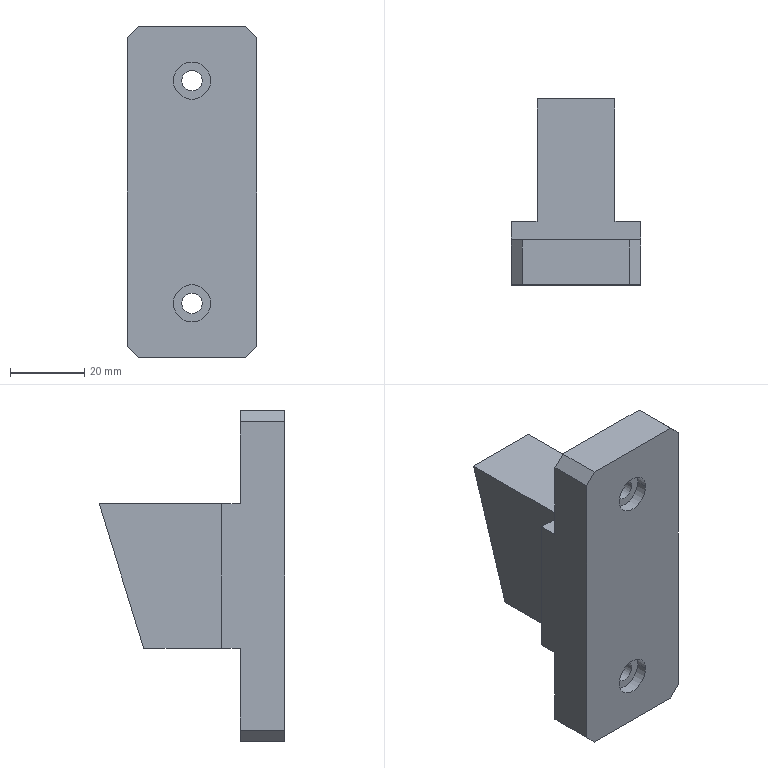Component | SolidWorks | QX1-15-PusherSlider-1 | 1 solid | 32 faces | box 35 x 50 x 89 mm | volume 64993 mm3 | plane 20 | cylinder 8 | cone 4 | commonest cylinder face diameters 5.5 x4 10 x4 | material PA Type 6
build123d program:
from build123d import *

# Parameters (mm, degrees)
BOSS_EXTRUDE1_DEPTH                                  = 17.5
SKETCH2_W                                            = 89
SKETCH2_H                                            = 12
BOSS_EXTRUDE2_DEPTH                                  = 35
SKETCH3_R                                            = 5
CUT_EXTRUDE1_DEPTH                                   = 3
CONICAL_COUNTERSUNK_HOLE1_FOR_M5_HEXAGON_D           = 5.5
CONICAL_COUNTERSUNK_HOLE1_FOR_M5_HEXAGON_CSINK_D     = 11.47
CONICAL_COUNTERSUNK_HOLE1_FOR_M5_HEXAGON_CSINK_ANGLE = 90
SKETCH7_W                                            = 39
SKETCH7_H                                            = 33
CUT_EXTRUDE2_DEPTH                                   = 7
CHAMFER1_SIZE                                        = 3


with BuildPart() as part:
    # Sketch1 → Boss-Extrude1 (new, symmetric)
    with BuildSketch(Plane.XY):
        Polygon((0, 0), (0, 38), (39, 50), (39, 0), align=None)
    extrude(amount=BOSS_EXTRUDE1_DEPTH, both=True)

    # Sketch2 → Boss-Extrude2 (add)
    with BuildSketch(Plane.XY.offset(17.5)):
        with Locations((19.5, 6)):
            Rectangle(SKETCH2_W, SKETCH2_H)
    extrude(amount=-BOSS_EXTRUDE2_DEPTH)

    # Sketch3 → Cut-Extrude1 (cut)
    with BuildSketch(Plane.XZ):
        with Locations(Location((-10.5, 0, 0), (0, 0, 270))):
            Circle(SKETCH3_R)
        with Locations(Location((49.5, 0, 0), (0, 0, 270))):
            Circle(SKETCH3_R)
    extrude(amount=-CUT_EXTRUDE1_DEPTH, mode=Mode.SUBTRACT)

    # Conical Countersunk Hole1 for M5 Hexagon (through all)
    with Locations(Plane(origin=(0, 12, 0), x_dir=(1, 0, 0), z_dir=(0, 1, 0))):
        with Locations((-10.5, 0), (49.5, 0)):
            CounterSinkHole(CONICAL_COUNTERSUNK_HOLE1_FOR_M5_HEXAGON_D / 2, CONICAL_COUNTERSUNK_HOLE1_FOR_M5_HEXAGON_CSINK_D / 2, counter_sink_angle=CONICAL_COUNTERSUNK_HOLE1_FOR_M5_HEXAGON_CSINK_ANGLE)

    # Sketch7 → Cut-Extrude2 (cut)
    with BuildSketch(Plane.XY.offset(17.5)):
        with Locations((19.5, 33.5)):
            Rectangle(SKETCH7_W, SKETCH7_H)
    cut_extrude2 = extrude(amount=-CUT_EXTRUDE2_DEPTH, mode=Mode.SUBTRACT)

    # Mirror1: Cut-Extrude2 across plane
    add(cut_extrude2.mirror(Plane.XY), mode=Mode.SUBTRACT)

    # Chamfer1
    chamfer1_edges = [part.edges().sort_by_distance(p)[0] for p in [
        (64, 6, 17.5),
        (-25, 6, 17.5),
        (-25, 6, -17.5),
        (64, 6, -17.5),
    ]]
    chamfer(chamfer1_edges, length=CHAMFER1_SIZE)


solid = part.part

# Placed as in the assembly
solid = solid.moved(Location((0, 40, -19.5), (0, -90, 0)))
STEP:
#1=COLOUR_RGB('',0.7922,0.8196,0.9333);
#2=FILL_AREA_STYLE_COLOUR('',#1);
#3=FILL_AREA_STYLE('',(#2));
#4=SURFACE_STYLE_FILL_AREA(#3);
#5=SURFACE_SIDE_STYLE('',(#4));
#6=SURFACE_STYLE_USAGE(.BOTH.,#5);
#7=PRESENTATION_STYLE_ASSIGNMENT((#6));
#8=CARTESIAN_POINT('',(0.1083,1.93,-1.181));
#9=VERTEX_POINT('',#8);
#10=CARTESIAN_POINT('',(-0.1083,1.93,-1.181));
#11=VERTEX_POINT('',#10);
#12=CARTESIAN_POINT('',(0.,1.93,-1.181));
#13=DIRECTION('',(-0.,1.,-0.));
#14=DIRECTION('',(-1.,-0.,0.));
#15=AXIS2_PLACEMENT_3D('',#12,#13,#14);
#16=CIRCLE('',#15,0.1083);
#17=EDGE_CURVE('',#9,#11,#16,.T.);
#18=ORIENTED_EDGE('',*,*,#17,.F.);
#19=CARTESIAN_POINT('',(0.2258,2.047,-1.181));
#20=VERTEX_POINT('',#19);
#21=CARTESIAN_POINT('',(0.2258,2.047,-1.181));
#22=DIRECTION('',(0.7071,0.7071,0.));
#23=VECTOR('',#22,39.37);
#24=LINE('',#21,#23);
#25=EDGE_CURVE('',#9,#20,#24,.T.);
#26=ORIENTED_EDGE('',*,*,#25,.T.);
#27=CARTESIAN_POINT('',(-0.2258,2.047,-1.181));
#28=VERTEX_POINT('',#27);
#29=CARTESIAN_POINT('',(0.,2.047,-1.181));
#30=DIRECTION('',(-0.,1.,-0.));
#31=DIRECTION('',(-1.,-0.,0.));
#32=AXIS2_PLACEMENT_3D('',#29,#30,#31);
#33=CIRCLE('',#32,0.2258);
#34=EDGE_CURVE('',#20,#28,#33,.T.);
#35=ORIENTED_EDGE('',*,*,#34,.T.);
#36=CARTESIAN_POINT('',(-0.2258,2.047,-1.181));
#37=DIRECTION('',(-0.7071,0.7071,-0.));
#38=VECTOR('',#37,39.37);
#39=LINE('',#36,#38);
#40=EDGE_CURVE('',#11,#28,#39,.T.);
#41=ORIENTED_EDGE('',*,*,#40,.F.);
#42=EDGE_LOOP('',(#18,#26,#35,#41));
#43=FACE_OUTER_BOUND('',#42,.T.);
#44=CARTESIAN_POINT('',(0.,2.047,-1.181));
#45=DIRECTION('',(-0.,1.,-0.));
#46=DIRECTION('',(-1.,-0.,0.));
#47=AXIS2_PLACEMENT_3D('',#44,#45,#46);
#48=CONICAL_SURFACE('',#47,0.2258,0.7854);
#49=ADVANCED_FACE('',(#43),#48,.F.);
#50=CARTESIAN_POINT('',(-0.1083,1.693,-1.181));
#51=VERTEX_POINT('',#50);
#52=CARTESIAN_POINT('',(0.1083,1.693,-1.181));
#53=VERTEX_POINT('',#52);
#54=CARTESIAN_POINT('',(0.,1.693,-1.181));
#55=DIRECTION('',(0.,-1.,0.));
#56=DIRECTION('',(1.,0.,0.));
#57=AXIS2_PLACEMENT_3D('',#54,#55,#56);
#58=CIRCLE('',#57,0.1083);
#59=EDGE_CURVE('',#51,#53,#58,.T.);
#60=ORIENTED_EDGE('',*,*,#59,.T.);
#61=CARTESIAN_POINT('',(0.1083,2.047,-1.181));
#62=DIRECTION('',(-0.,1.,-0.));
#63=VECTOR('',#62,39.37);
#64=LINE('',#61,#63);
#65=EDGE_CURVE('',#53,#9,#64,.T.);
#66=ORIENTED_EDGE('',*,*,#65,.T.);
#67=ORIENTED_EDGE('',*,*,#17,.T.);
#68=CARTESIAN_POINT('',(-0.1083,2.047,-1.181));
#69=DIRECTION('',(-0.,1.,-0.));
#70=VECTOR('',#69,39.37);
#71=LINE('',#68,#70);
#72=EDGE_CURVE('',#51,#11,#71,.T.);
#73=ORIENTED_EDGE('',*,*,#72,.F.);
#74=EDGE_LOOP('',(#60,#66,#67,#73));
#75=FACE_OUTER_BOUND('',#74,.T.);
#76=CARTESIAN_POINT('',(0.,2.047,-1.181));
#77=DIRECTION('',(-0.,1.,-0.));
#78=DIRECTION('',(-1.,-0.,0.));
#79=AXIS2_PLACEMENT_3D('',#76,#77,#78);
#80=CYLINDRICAL_SURFACE('',#79,0.1083);
#81=ADVANCED_FACE('',(#75),#80,.F.);
#82=CARTESIAN_POINT('',(0.1083,1.93,1.181));
#83=VERTEX_POINT('',#82);
#84=CARTESIAN_POINT('',(-0.1083,1.93,1.181));
#85=VERTEX_POINT('',#84);
#86=CARTESIAN_POINT('',(0.,1.93,1.181));
#87=DIRECTION('',(-0.,1.,-0.));
#88=DIRECTION('',(-1.,-0.,0.));
#89=AXIS2_PLACEMENT_3D('',#86,#87,#88);
#90=CIRCLE('',#89,0.1083);
#91=EDGE_CURVE('',#83,#85,#90,.T.);
#92=ORIENTED_EDGE('',*,*,#91,.F.);
#93=CARTESIAN_POINT('',(0.2258,2.047,1.181));
#94=VERTEX_POINT('',#93);
#95=CARTESIAN_POINT('',(0.2258,2.047,1.181));
#96=DIRECTION('',(0.7071,0.7071,0.));
#97=VECTOR('',#96,39.37);
#98=LINE('',#95,#97);
#99=EDGE_CURVE('',#83,#94,#98,.T.);
#100=ORIENTED_EDGE('',*,*,#99,.T.);
#101=CARTESIAN_POINT('',(-0.2258,2.047,1.181));
#102=VERTEX_POINT('',#101);
#103=CARTESIAN_POINT('',(0.,2.047,1.181));
#104=DIRECTION('',(-0.,1.,-0.));
#105=DIRECTION('',(-1.,-0.,0.));
#106=AXIS2_PLACEMENT_3D('',#103,#104,#105);
#107=CIRCLE('',#106,0.2258);
#108=EDGE_CURVE('',#94,#102,#107,.T.);
#109=ORIENTED_EDGE('',*,*,#108,.T.);
#110=CARTESIAN_POINT('',(-0.2258,2.047,1.181));
#111=DIRECTION('',(-0.7071,0.7071,-0.));
#112=VECTOR('',#111,39.37);
#113=LINE('',#110,#112);
#114=EDGE_CURVE('',#85,#102,#113,.T.);
#115=ORIENTED_EDGE('',*,*,#114,.F.);
#116=EDGE_LOOP('',(#92,#100,#109,#115));
#117=FACE_OUTER_BOUND('',#116,.T.);
#118=CARTESIAN_POINT('',(0.,2.047,1.181));
#119=DIRECTION('',(-0.,1.,-0.));
#120=DIRECTION('',(-1.,-0.,0.));
#121=AXIS2_PLACEMENT_3D('',#118,#119,#120);
#122=CONICAL_SURFACE('',#121,0.2258,0.7854);
#123=ADVANCED_FACE('',(#117),#122,.F.);
#124=CARTESIAN_POINT('',(-0.1083,1.693,1.181));
#125=VERTEX_POINT('',#124);
#126=CARTESIAN_POINT('',(0.1083,1.693,1.181));
#127=VERTEX_POINT('',#126);
#128=CARTESIAN_POINT('',(0.,1.693,1.181));
#129=DIRECTION('',(0.,-1.,0.));
#130=DIRECTION('',(1.,0.,0.));
#131=AXIS2_PLACEMENT_3D('',#128,#129,#130);
#132=CIRCLE('',#131,0.1083);
#133=EDGE_CURVE('',#125,#127,#132,.T.);
#134=ORIENTED_EDGE('',*,*,#133,.T.);
#135=CARTESIAN_POINT('',(0.1083,2.047,1.181));
#136=DIRECTION('',(-0.,1.,-0.));
#137=VECTOR('',#136,39.37);
#138=LINE('',#135,#137);
#139=EDGE_CURVE('',#127,#83,#138,.T.);
#140=ORIENTED_EDGE('',*,*,#139,.T.);
#141=ORIENTED_EDGE('',*,*,#91,.T.);
#142=CARTESIAN_POINT('',(-0.1083,2.047,1.181));
#143=DIRECTION('',(-0.,1.,-0.));
#144=VECTOR('',#143,39.37);
#145=LINE('',#142,#144);
#146=EDGE_CURVE('',#125,#85,#145,.T.);
#147=ORIENTED_EDGE('',*,*,#146,.F.);
#148=EDGE_LOOP('',(#134,#140,#141,#147));
#149=FACE_OUTER_BOUND('',#148,.T.);
#150=CARTESIAN_POINT('',(0.,2.047,1.181));
#151=DIRECTION('',(-0.,1.,-0.));
#152=DIRECTION('',(-1.,-0.,0.));
#153=AXIS2_PLACEMENT_3D('',#150,#151,#152);
#154=CYLINDRICAL_SURFACE('',#153,0.1083);
#155=ADVANCED_FACE('',(#149),#154,.F.);
#156=CARTESIAN_POINT('',(-0.1969,1.693,-1.181));
#157=VERTEX_POINT('',#156);
#158=CARTESIAN_POINT('',(0.1969,1.693,-1.181));
#159=VERTEX_POINT('',#158);
#160=CARTESIAN_POINT('',(0.,1.693,-1.181));
#161=DIRECTION('',(0.,-1.,0.));
#162=DIRECTION('',(1.,0.,0.));
#163=AXIS2_PLACEMENT_3D('',#160,#161,#162);
#164=CIRCLE('',#163,0.1969);
#165=EDGE_CURVE('',#157,#159,#164,.T.);
#166=ORIENTED_EDGE('',*,*,#165,.F.);
#167=CARTESIAN_POINT('',(-0.1969,1.575,-1.181));
#168=VERTEX_POINT('',#167);
#169=CARTESIAN_POINT('',(-0.1969,1.693,-1.181));
#170=DIRECTION('',(0.,-1.,0.));
#171=VECTOR('',#170,39.37);
#172=LINE('',#169,#171);
#173=EDGE_CURVE('',#157,#168,#172,.T.);
#174=ORIENTED_EDGE('',*,*,#173,.T.);
#175=CARTESIAN_POINT('',(0.1969,1.575,-1.181));
#176=VERTEX_POINT('',#175);
#177=CARTESIAN_POINT('',(0.,1.575,-1.181));
#178=DIRECTION('',(0.,-1.,0.));
#179=DIRECTION('',(1.,0.,0.));
#180=AXIS2_PLACEMENT_3D('',#177,#178,#179);
#181=CIRCLE('',#180,0.1969);
#182=EDGE_CURVE('',#168,#176,#181,.T.);
#183=ORIENTED_EDGE('',*,*,#182,.T.);
#184=CARTESIAN_POINT('',(0.1969,1.693,-1.181));
#185=DIRECTION('',(0.,-1.,0.));
#186=VECTOR('',#185,39.37);
#187=LINE('',#184,#186);
#188=EDGE_CURVE('',#159,#176,#187,.T.);
#189=ORIENTED_EDGE('',*,*,#188,.F.);
#190=EDGE_LOOP('',(#166,#174,#183,#189));
#191=FACE_OUTER_BOUND('',#190,.T.);
#192=CARTESIAN_POINT('',(0.,1.693,-1.181));
#193=DIRECTION('',(0.,-1.,0.));
#194=DIRECTION('',(1.,0.,0.));
#195=AXIS2_PLACEMENT_3D('',#192,#193,#194);
#196=CYLINDRICAL_SURFACE('',#195,0.1969);
#197=ADVANCED_FACE('',(#191),#196,.F.);
#198=CARTESIAN_POINT('',(-0.1969,1.693,1.181));
#199=VERTEX_POINT('',#198);
#200=CARTESIAN_POINT('',(0.1969,1.693,1.181));
#201=VERTEX_POINT('',#200);
#202=CARTESIAN_POINT('',(0.,1.693,1.181));
#203=DIRECTION('',(0.,-1.,0.));
#204=DIRECTION('',(1.,0.,0.));
#205=AXIS2_PLACEMENT_3D('',#202,#203,#204);
#206=CIRCLE('',#205,0.1969);
#207=EDGE_CURVE('',#199,#201,#206,.T.);
#208=ORIENTED_EDGE('',*,*,#207,.F.);
#209=CARTESIAN_POINT('',(-0.1969,1.575,1.181));
#210=VERTEX_POINT('',#209);
#211=CARTESIAN_POINT('',(-0.1969,1.693,1.181));
#212=DIRECTION('',(0.,-1.,0.));
#213=VECTOR('',#212,39.37);
#214=LINE('',#211,#213);
#215=EDGE_CURVE('',#199,#210,#214,.T.);
#216=ORIENTED_EDGE('',*,*,#215,.T.);
#217=CARTESIAN_POINT('',(0.1969,1.575,1.181));
#218=VERTEX_POINT('',#217);
#219=CARTESIAN_POINT('',(0.,1.575,1.181));
#220=DIRECTION('',(0.,-1.,0.));
#221=DIRECTION('',(1.,0.,0.));
#222=AXIS2_PLACEMENT_3D('',#219,#220,#221);
#223=CIRCLE('',#222,0.1969);
#224=EDGE_CURVE('',#210,#218,#223,.T.);
#225=ORIENTED_EDGE('',*,*,#224,.T.);
#226=CARTESIAN_POINT('',(0.1969,1.693,1.181));
#227=DIRECTION('',(0.,-1.,0.));
#228=VECTOR('',#227,39.37);
#229=LINE('',#226,#228);
#230=EDGE_CURVE('',#201,#218,#229,.T.);
#231=ORIENTED_EDGE('',*,*,#230,.F.);
#232=EDGE_LOOP('',(#208,#216,#225,#231));
#233=FACE_OUTER_BOUND('',#232,.T.);
#234=CARTESIAN_POINT('',(0.,1.693,1.181));
#235=DIRECTION('',(0.,-1.,0.));
#236=DIRECTION('',(1.,0.,0.));
#237=AXIS2_PLACEMENT_3D('',#234,#235,#236);
#238=CYLINDRICAL_SURFACE('',#237,0.1969);
#239=ADVANCED_FACE('',(#233),#238,.F.);
#240=CARTESIAN_POINT('',(0.4134,3.071,-0.7677));
#241=VERTEX_POINT('',#240);
#242=CARTESIAN_POINT('',(0.4134,3.543,0.7677));
#243=VERTEX_POINT('',#242);
#244=CARTESIAN_POINT('',(0.4134,3.071,-0.7677));
#245=DIRECTION('',(-0.,0.2941,0.9558));
#246=VECTOR('',#245,39.37);
#247=LINE('',#244,#246);
#248=EDGE_CURVE('',#241,#243,#247,.T.);
#249=ORIENTED_EDGE('',*,*,#248,.F.);
#250=CARTESIAN_POINT('',(-0.4134,3.071,-0.7677));
#251=VERTEX_POINT('',#250);
#252=CARTESIAN_POINT('',(-0.689,3.071,-0.7677));
#253=DIRECTION('',(1.,0.,0.));
#254=VECTOR('',#253,39.37);
#255=LINE('',#252,#254);
#256=EDGE_CURVE('',#251,#241,#255,.T.);
#257=ORIENTED_EDGE('',*,*,#256,.F.);
#258=CARTESIAN_POINT('',(-0.4134,3.543,0.7677));
#259=VERTEX_POINT('',#258);
#260=CARTESIAN_POINT('',(-0.4134,3.071,-0.7677));
#261=DIRECTION('',(0.,-0.2941,-0.9558));
#262=VECTOR('',#261,39.37);
#263=LINE('',#260,#262);
#264=EDGE_CURVE('',#259,#251,#263,.T.);
#265=ORIENTED_EDGE('',*,*,#264,.F.);
#266=CARTESIAN_POINT('',(-0.689,3.543,0.7677));
#267=DIRECTION('',(1.,0.,0.));
#268=VECTOR('',#267,39.37);
#269=LINE('',#266,#268);
#270=EDGE_CURVE('',#259,#243,#269,.T.);
#271=ORIENTED_EDGE('',*,*,#270,.T.);
#272=EDGE_LOOP('',(#249,#257,#265,#271));
#273=FACE_OUTER_BOUND('',#272,.T.);
#274=CARTESIAN_POINT('',(-0.689,3.071,-0.7677));
#275=DIRECTION('',(0.,-0.9558,0.2941));
#276=DIRECTION('',(-0.,0.2941,0.9558));
#277=AXIS2_PLACEMENT_3D('',#274,#275,#276);
#278=PLANE('',#277);
#279=ADVANCED_FACE('',(#273),#278,.F.);
#280=CARTESIAN_POINT('',(0.4134,2.244,0.7677));
#281=VERTEX_POINT('',#280);
#282=CARTESIAN_POINT('',(0.689,2.244,0.7677));
#283=VERTEX_POINT('',#282);
#284=CARTESIAN_POINT('',(0.4134,2.244,0.7677));
#285=DIRECTION('',(1.,0.,0.));
#286=VECTOR('',#285,39.37);
#287=LINE('',#284,#286);
#288=EDGE_CURVE('',#281,#283,#287,.T.);
#289=ORIENTED_EDGE('',*,*,#288,.F.);
#290=CARTESIAN_POINT('',(0.4134,3.543,0.7677));
#291=DIRECTION('',(-0.,1.,-0.));
#292=VECTOR('',#291,39.37);
#293=LINE('',#290,#292);
#294=EDGE_CURVE('',#281,#243,#293,.T.);
#295=ORIENTED_EDGE('',*,*,#294,.T.);
#296=ORIENTED_EDGE('',*,*,#270,.F.);
#297=CARTESIAN_POINT('',(-0.4134,2.244,0.7677));
#298=VERTEX_POINT('',#297);
#299=CARTESIAN_POINT('',(-0.4134,3.543,0.7677));
#300=DIRECTION('',(-0.,1.,-0.));
#301=VECTOR('',#300,39.37);
#302=LINE('',#299,#301);
#303=EDGE_CURVE('',#298,#259,#302,.T.);
#304=ORIENTED_EDGE('',*,*,#303,.F.);
#305=CARTESIAN_POINT('',(-0.689,2.244,0.7677));
#306=VERTEX_POINT('',#305);
#307=CARTESIAN_POINT('',(-0.4134,2.244,0.7677));
#308=DIRECTION('',(-1.,-0.,-0.));
#309=VECTOR('',#308,39.37);
#310=LINE('',#307,#309);
#311=EDGE_CURVE('',#298,#306,#310,.T.);
#312=ORIENTED_EDGE('',*,*,#311,.T.);
#313=CARTESIAN_POINT('',(-0.689,2.047,0.7677));
#314=VERTEX_POINT('',#313);
#315=CARTESIAN_POINT('',(-0.689,3.543,0.7677));
#316=DIRECTION('',(-0.,1.,-0.));
#317=VECTOR('',#316,39.37);
#318=LINE('',#315,#317);
#319=EDGE_CURVE('',#314,#306,#318,.T.);
#320=ORIENTED_EDGE('',*,*,#319,.F.);
#321=CARTESIAN_POINT('',(0.689,2.047,0.7677));
#322=VERTEX_POINT('',#321);
#323=CARTESIAN_POINT('',(-0.689,2.047,0.7677));
#324=DIRECTION('',(1.,0.,0.));
#325=VECTOR('',#324,39.37);
#326=LINE('',#323,#325);
#327=EDGE_CURVE('',#314,#322,#326,.T.);
#328=ORIENTED_EDGE('',*,*,#327,.T.);
#329=CARTESIAN_POINT('',(0.689,3.543,0.7677));
#330=DIRECTION('',(-0.,1.,-0.));
#331=VECTOR('',#330,39.37);
#332=LINE('',#329,#331);
#333=EDGE_CURVE('',#322,#283,#332,.T.);
#334=ORIENTED_EDGE('',*,*,#333,.T.);
#335=EDGE_LOOP('',(#289,#295,#296,#304,#312,#320,#328,#334));
#336=FACE_OUTER_BOUND('',#335,.T.);
#337=CARTESIAN_POINT('',(-0.689,3.543,0.7677));
#338=DIRECTION('',(0.,-0.,-1.));
#339=DIRECTION('',(0.,-1.,0.));
#340=AXIS2_PLACEMENT_3D('',#337,#338,#339);
#341=PLANE('',#340);
#342=ADVANCED_FACE('',(#336),#341,.F.);
#343=CARTESIAN_POINT('',(0.4134,2.244,-0.7677));
#344=VERTEX_POINT('',#343);
#345=CARTESIAN_POINT('',(0.689,2.244,-0.7677));
#346=VERTEX_POINT('',#345);
#347=CARTESIAN_POINT('',(0.4134,2.244,-0.7677));
#348=DIRECTION('',(1.,0.,0.));
#349=VECTOR('',#348,39.37);
#350=LINE('',#347,#349);
#351=EDGE_CURVE('',#344,#346,#350,.T.);
#352=ORIENTED_EDGE('',*,*,#351,.T.);
#353=CARTESIAN_POINT('',(0.689,2.047,-0.7677));
#354=VERTEX_POINT('',#353);
#355=CARTESIAN_POINT('',(0.689,1.575,-0.7677));
#356=DIRECTION('',(0.,-1.,0.));
#357=VECTOR('',#356,39.37);
#358=LINE('',#355,#357);
#359=EDGE_CURVE('',#346,#354,#358,.T.);
#360=ORIENTED_EDGE('',*,*,#359,.T.);
#361=CARTESIAN_POINT('',(-0.689,2.047,-0.7677));
#362=VERTEX_POINT('',#361);
#363=CARTESIAN_POINT('',(-0.689,2.047,-0.7677));
#364=DIRECTION('',(-1.,-0.,-0.));
#365=VECTOR('',#364,39.37);
#366=LINE('',#363,#365);
#367=EDGE_CURVE('',#354,#362,#366,.T.);
#368=ORIENTED_EDGE('',*,*,#367,.T.);
#369=CARTESIAN_POINT('',(-0.689,2.244,-0.7677));
#370=VERTEX_POINT('',#369);
#371=CARTESIAN_POINT('',(-0.689,1.575,-0.7677));
#372=DIRECTION('',(0.,-1.,0.));
#373=VECTOR('',#372,39.37);
#374=LINE('',#371,#373);
#375=EDGE_CURVE('',#370,#362,#374,.T.);
#376=ORIENTED_EDGE('',*,*,#375,.F.);
#377=CARTESIAN_POINT('',(-0.4134,2.244,-0.7677));
#378=VERTEX_POINT('',#377);
#379=CARTESIAN_POINT('',(-0.4134,2.244,-0.7677));
#380=DIRECTION('',(-1.,-0.,-0.));
#381=VECTOR('',#380,39.37);
#382=LINE('',#379,#381);
#383=EDGE_CURVE('',#378,#370,#382,.T.);
#384=ORIENTED_EDGE('',*,*,#383,.F.);
#385=CARTESIAN_POINT('',(-0.4134,3.543,-0.7677));
#386=DIRECTION('',(0.,-1.,0.));
#387=VECTOR('',#386,39.37);
#388=LINE('',#385,#387);
#389=EDGE_CURVE('',#251,#378,#388,.T.);
#390=ORIENTED_EDGE('',*,*,#389,.F.);
#391=ORIENTED_EDGE('',*,*,#256,.T.);
#392=CARTESIAN_POINT('',(0.4134,3.543,-0.7677));
#393=DIRECTION('',(0.,-1.,0.));
#394=VECTOR('',#393,39.37);
#395=LINE('',#392,#394);
#396=EDGE_CURVE('',#241,#344,#395,.T.);
#397=ORIENTED_EDGE('',*,*,#396,.T.);
#398=EDGE_LOOP('',(#352,#360,#368,#376,#384,#390,#391,#397));
#399=FACE_OUTER_BOUND('',#398,.T.);
#400=CARTESIAN_POINT('',(-0.689,1.575,-0.7677));
#401=DIRECTION('',(-0.,0.,1.));
#402=DIRECTION('',(1.,0.,0.));
#403=AXIS2_PLACEMENT_3D('',#400,#401,#402);
#404=PLANE('',#403);
#405=ADVANCED_FACE('',(#399),#404,.F.);
#406=CARTESIAN_POINT('',(0.689,2.047,1.634));
#407=VERTEX_POINT('',#406);
#408=CARTESIAN_POINT('',(0.689,2.047,-1.752));
#409=DIRECTION('',(0.,-0.,-1.));
#410=VECTOR('',#409,39.37);
#411=LINE('',#408,#410);
#412=EDGE_CURVE('',#407,#322,#411,.T.);
#413=ORIENTED_EDGE('',*,*,#412,.F.);
#414=CARTESIAN_POINT('',(0.689,1.575,1.634));
#415=VERTEX_POINT('',#414);
#416=CARTESIAN_POINT('',(0.689,1.575,1.634));
#417=DIRECTION('',(0.,-1.,0.));
#418=VECTOR('',#417,39.37);
#419=LINE('',#416,#418);
#420=EDGE_CURVE('',#407,#415,#419,.T.);
#421=ORIENTED_EDGE('',*,*,#420,.T.);
#422=CARTESIAN_POINT('',(0.689,1.575,-1.634));
#423=VERTEX_POINT('',#422);
#424=CARTESIAN_POINT('',(0.689,1.575,0.7677));
#425=DIRECTION('',(-0.,0.,1.));
#426=VECTOR('',#425,39.37);
#427=LINE('',#424,#426);
#428=EDGE_CURVE('',#423,#415,#427,.T.);
#429=ORIENTED_EDGE('',*,*,#428,.F.);
#430=CARTESIAN_POINT('',(0.689,2.047,-1.634));
#431=VERTEX_POINT('',#430);
#432=CARTESIAN_POINT('',(0.689,1.575,-1.634));
#433=DIRECTION('',(-0.,1.,-0.));
#434=VECTOR('',#433,39.37);
#435=LINE('',#432,#434);
#436=EDGE_CURVE('',#423,#431,#435,.T.);
#437=ORIENTED_EDGE('',*,*,#436,.T.);
#438=CARTESIAN_POINT('',(0.689,2.047,-1.752));
#439=DIRECTION('',(0.,-0.,-1.));
#440=VECTOR('',#439,39.37);
#441=LINE('',#438,#440);
#442=EDGE_CURVE('',#354,#431,#441,.T.);
#443=ORIENTED_EDGE('',*,*,#442,.F.);
#444=ORIENTED_EDGE('',*,*,#359,.F.);
#445=CARTESIAN_POINT('',(0.689,2.244,-0.7677));
#446=DIRECTION('',(-0.,0.,1.));
#447=VECTOR('',#446,39.37);
#448=LINE('',#445,#447);
#449=EDGE_CURVE('',#346,#283,#448,.T.);
#450=ORIENTED_EDGE('',*,*,#449,.T.);
#451=ORIENTED_EDGE('',*,*,#333,.F.);
#452=EDGE_LOOP('',(#413,#421,#429,#437,#443,#444,#450,#451));
#453=FACE_OUTER_BOUND('',#452,.T.);
#454=CARTESIAN_POINT('',(0.689,1.575,-0.7677));
#455=DIRECTION('',(1.,0.,0.));
#456=DIRECTION('',(0.,-0.,-1.));
#457=AXIS2_PLACEMENT_3D('',#454,#455,#456);
#458=PLANE('',#457);
#459=ADVANCED_FACE('',(#453),#458,.T.);
#460=CARTESIAN_POINT('',(0.,1.575,-1.181));
#461=DIRECTION('',(0.,-1.,0.));
#462=DIRECTION('',(1.,0.,0.));
#463=AXIS2_PLACEMENT_3D('',#460,#461,#462);
#464=CIRCLE('',#463,0.1969);
#465=EDGE_CURVE('',#176,#168,#464,.T.);
#466=ORIENTED_EDGE('',*,*,#465,.F.);
#467=ORIENTED_EDGE('',*,*,#182,.F.);
#468=EDGE_LOOP('',(#466,#467));
#469=FACE_BOUND('',#468,.T.);
#470=CARTESIAN_POINT('',(0.,1.575,1.181));
#471=DIRECTION('',(0.,-1.,0.));
#472=DIRECTION('',(1.,0.,0.));
#473=AXIS2_PLACEMENT_3D('',#470,#471,#472);
#474=CIRCLE('',#473,0.1969);
#475=EDGE_CURVE('',#218,#210,#474,.T.);
#476=ORIENTED_EDGE('',*,*,#475,.F.);
#477=ORIENTED_EDGE('',*,*,#224,.F.);
#478=EDGE_LOOP('',(#476,#477));
#479=FACE_BOUND('',#478,.T.);
#480=ORIENTED_EDGE('',*,*,#428,.T.);
#481=CARTESIAN_POINT('',(0.5709,1.575,1.752));
#482=VERTEX_POINT('',#481);
#483=CARTESIAN_POINT('',(0.5709,1.575,1.752));
#484=DIRECTION('',(-0.7071,-0.,0.7071));
#485=VECTOR('',#484,39.37);
#486=LINE('',#483,#485);
#487=EDGE_CURVE('',#415,#482,#486,.T.);
#488=ORIENTED_EDGE('',*,*,#487,.T.);
#489=CARTESIAN_POINT('',(-0.5709,1.575,1.752));
#490=VERTEX_POINT('',#489);
#491=CARTESIAN_POINT('',(0.689,1.575,1.752));
#492=DIRECTION('',(-1.,-0.,-0.));
#493=VECTOR('',#492,39.37);
#494=LINE('',#491,#493);
#495=EDGE_CURVE('',#482,#490,#494,.T.);
#496=ORIENTED_EDGE('',*,*,#495,.T.);
#497=CARTESIAN_POINT('',(-0.689,1.575,1.634));
#498=VERTEX_POINT('',#497);
#499=CARTESIAN_POINT('',(-0.689,1.575,1.634));
#500=DIRECTION('',(-0.7071,-0.,-0.7071));
#501=VECTOR('',#500,39.37);
#502=LINE('',#499,#501);
#503=EDGE_CURVE('',#490,#498,#502,.T.);
#504=ORIENTED_EDGE('',*,*,#503,.T.);
#505=CARTESIAN_POINT('',(-0.689,1.575,-1.634));
#506=VERTEX_POINT('',#505);
#507=CARTESIAN_POINT('',(-0.689,1.575,0.7677));
#508=DIRECTION('',(-0.,0.,1.));
#509=VECTOR('',#508,39.37);
#510=LINE('',#507,#509);
#511=EDGE_CURVE('',#506,#498,#510,.T.);
#512=ORIENTED_EDGE('',*,*,#511,.F.);
#513=CARTESIAN_POINT('',(-0.5709,1.575,-1.752));
#514=VERTEX_POINT('',#513);
#515=CARTESIAN_POINT('',(-0.689,1.575,-1.634));
#516=DIRECTION('',(0.7071,0.,-0.7071));
#517=VECTOR('',#516,39.37);
#518=LINE('',#515,#517);
#519=EDGE_CURVE('',#506,#514,#518,.T.);
#520=ORIENTED_EDGE('',*,*,#519,.T.);
#521=CARTESIAN_POINT('',(0.5709,1.575,-1.752));
#522=VERTEX_POINT('',#521);
#523=CARTESIAN_POINT('',(0.689,1.575,-1.752));
#524=DIRECTION('',(-1.,-0.,-0.));
#525=VECTOR('',#524,39.37);
#526=LINE('',#523,#525);
#527=EDGE_CURVE('',#522,#514,#526,.T.);
#528=ORIENTED_EDGE('',*,*,#527,.F.);
#529=CARTESIAN_POINT('',(0.5709,1.575,-1.752));
#530=DIRECTION('',(0.7071,0.,0.7071));
#531=VECTOR('',#530,39.37);
#532=LINE('',#529,#531);
#533=EDGE_CURVE('',#522,#423,#532,.T.);
#534=ORIENTED_EDGE('',*,*,#533,.T.);
#535=EDGE_LOOP('',(#480,#488,#496,#504,#512,#520,#528,#534));
#536=FACE_OUTER_BOUND('',#535,.T.);
#537=CARTESIAN_POINT('',(-0.689,1.575,0.7677));
#538=DIRECTION('',(-0.,1.,-0.));
#539=DIRECTION('',(-1.,-0.,-0.));
#540=AXIS2_PLACEMENT_3D('',#537,#538,#539);
#541=PLANE('',#540);
#542=ADVANCED_FACE('',(#469,#479,#536),#541,.F.);
#543=ORIENTED_EDGE('',*,*,#511,.T.);
#544=CARTESIAN_POINT('',(-0.689,2.047,1.634));
#545=VERTEX_POINT('',#544);
#546=CARTESIAN_POINT('',(-0.689,2.047,1.634));
#547=DIRECTION('',(-0.,1.,-0.));
#548=VECTOR('',#547,39.37);
#549=LINE('',#546,#548);
#550=EDGE_CURVE('',#498,#545,#549,.T.);
#551=ORIENTED_EDGE('',*,*,#550,.T.);
#552=CARTESIAN_POINT('',(-0.689,2.047,-1.752));
#553=DIRECTION('',(0.,-0.,-1.));
#554=VECTOR('',#553,39.37);
#555=LINE('',#552,#554);
#556=EDGE_CURVE('',#545,#314,#555,.T.);
#557=ORIENTED_EDGE('',*,*,#556,.T.);
#558=ORIENTED_EDGE('',*,*,#319,.T.);
#559=CARTESIAN_POINT('',(-0.689,2.244,-0.7677));
#560=DIRECTION('',(-0.,0.,1.));
#561=VECTOR('',#560,39.37);
#562=LINE('',#559,#561);
#563=EDGE_CURVE('',#370,#306,#562,.T.);
#564=ORIENTED_EDGE('',*,*,#563,.F.);
#565=ORIENTED_EDGE('',*,*,#375,.T.);
#566=CARTESIAN_POINT('',(-0.689,2.047,-1.634));
#567=VERTEX_POINT('',#566);
#568=CARTESIAN_POINT('',(-0.689,2.047,-1.752));
#569=DIRECTION('',(0.,-0.,-1.));
#570=VECTOR('',#569,39.37);
#571=LINE('',#568,#570);
#572=EDGE_CURVE('',#362,#567,#571,.T.);
#573=ORIENTED_EDGE('',*,*,#572,.T.);
#574=CARTESIAN_POINT('',(-0.689,1.575,-1.634));
#575=DIRECTION('',(0.,-1.,0.));
#576=VECTOR('',#575,39.37);
#577=LINE('',#574,#576);
#578=EDGE_CURVE('',#567,#506,#577,.T.);
#579=ORIENTED_EDGE('',*,*,#578,.T.);
#580=EDGE_LOOP('',(#543,#551,#557,#558,#564,#565,#573,#579));
#581=FACE_OUTER_BOUND('',#580,.T.);
#582=CARTESIAN_POINT('',(-0.689,1.575,-0.7677));
#583=DIRECTION('',(1.,0.,0.));
#584=DIRECTION('',(0.,-0.,-1.));
#585=AXIS2_PLACEMENT_3D('',#582,#583,#584);
#586=PLANE('',#585);
#587=ADVANCED_FACE('',(#581),#586,.F.);
#588=CARTESIAN_POINT('',(0.5709,2.047,-1.752));
#589=VERTEX_POINT('',#588);
#590=CARTESIAN_POINT('',(-0.5709,2.047,-1.752));
#591=VERTEX_POINT('',#590);
#592=CARTESIAN_POINT('',(0.689,2.047,-1.752));
#593=DIRECTION('',(-1.,-0.,-0.));
#594=VECTOR('',#593,39.37);
#595=LINE('',#592,#594);
#596=EDGE_CURVE('',#589,#591,#595,.T.);
#597=ORIENTED_EDGE('',*,*,#596,.F.);
#598=CARTESIAN_POINT('',(0.5709,1.575,-1.752));
#599=DIRECTION('',(0.,-1.,0.));
#600=VECTOR('',#599,39.37);
#601=LINE('',#598,#600);
#602=EDGE_CURVE('',#589,#522,#601,.T.);
#603=ORIENTED_EDGE('',*,*,#602,.T.);
#604=ORIENTED_EDGE('',*,*,#527,.T.);
#605=CARTESIAN_POINT('',(-0.5709,2.047,-1.752));
#606=DIRECTION('',(-0.,1.,-0.));
#607=VECTOR('',#606,39.37);
#608=LINE('',#605,#607);
#609=EDGE_CURVE('',#514,#591,#608,.T.);
#610=ORIENTED_EDGE('',*,*,#609,.T.);
#611=EDGE_LOOP('',(#597,#603,#604,#610));
#612=FACE_OUTER_BOUND('',#611,.T.);
#613=CARTESIAN_POINT('',(0.689,1.575,-1.752));
#614=DIRECTION('',(0.,-0.,-1.));
#615=DIRECTION('',(-1.,-0.,-0.));
#616=AXIS2_PLACEMENT_3D('',#613,#614,#615);
#617=PLANE('',#616);
#618=ADVANCED_FACE('',(#612),#617,.T.);
#619=CARTESIAN_POINT('',(0.,2.047,-1.181));
#620=DIRECTION('',(-0.,1.,-0.));
#621=DIRECTION('',(-1.,-0.,0.));
#622=AXIS2_PLACEMENT_3D('',#619,#620,#621);
#623=CIRCLE('',#622,0.2258);
#624=EDGE_CURVE('',#28,#20,#623,.T.);
#625=ORIENTED_EDGE('',*,*,#624,.F.);
#626=ORIENTED_EDGE('',*,*,#34,.F.);
#627=EDGE_LOOP('',(#625,#626));
#628=FACE_BOUND('',#627,.T.);
#629=ORIENTED_EDGE('',*,*,#442,.T.);
#630=CARTESIAN_POINT('',(0.6299,2.047,-1.693));
#631=DIRECTION('',(-0.7071,-0.,-0.7071));
#632=VECTOR('',#631,39.37);
#633=LINE('',#630,#632);
#634=EDGE_CURVE('',#431,#589,#633,.T.);
#635=ORIENTED_EDGE('',*,*,#634,.T.);
#636=ORIENTED_EDGE('',*,*,#596,.T.);
#637=CARTESIAN_POINT('',(0.05906,2.047,-2.382));
#638=DIRECTION('',(-0.7071,-0.,0.7071));
#639=VECTOR('',#638,39.37);
#640=LINE('',#637,#639);
#641=EDGE_CURVE('',#591,#567,#640,.T.);
#642=ORIENTED_EDGE('',*,*,#641,.T.);
#643=ORIENTED_EDGE('',*,*,#572,.F.);
#644=ORIENTED_EDGE('',*,*,#367,.F.);
#645=EDGE_LOOP('',(#629,#635,#636,#642,#643,#644));
#646=FACE_OUTER_BOUND('',#645,.T.);
#647=CARTESIAN_POINT('',(0.689,2.047,-1.752));
#648=DIRECTION('',(-0.,1.,-0.));
#649=DIRECTION('',(-1.,-0.,-0.));
#650=AXIS2_PLACEMENT_3D('',#647,#648,#649);
#651=PLANE('',#650);
#652=ADVANCED_FACE('',(#628,#646),#651,.T.);
#653=CARTESIAN_POINT('',(0.,2.047,1.181));
#654=DIRECTION('',(-0.,1.,-0.));
#655=DIRECTION('',(-1.,-0.,0.));
#656=AXIS2_PLACEMENT_3D('',#653,#654,#655);
#657=CIRCLE('',#656,0.2258);
#658=EDGE_CURVE('',#102,#94,#657,.T.);
#659=ORIENTED_EDGE('',*,*,#658,.F.);
#660=ORIENTED_EDGE('',*,*,#108,.F.);
#661=EDGE_LOOP('',(#659,#660));
#662=FACE_BOUND('',#661,.T.);
#663=CARTESIAN_POINT('',(0.5709,2.047,1.752));
#664=VERTEX_POINT('',#663);
#665=CARTESIAN_POINT('',(-0.5709,2.047,1.752));
#666=VERTEX_POINT('',#665);
#667=CARTESIAN_POINT('',(0.689,2.047,1.752));
#668=DIRECTION('',(-1.,-0.,-0.));
#669=VECTOR('',#668,39.37);
#670=LINE('',#667,#669);
#671=EDGE_CURVE('',#664,#666,#670,.T.);
#672=ORIENTED_EDGE('',*,*,#671,.F.);
#673=CARTESIAN_POINT('',(2.382,2.047,-0.05906));
#674=DIRECTION('',(0.7071,0.,-0.7071));
#675=VECTOR('',#674,39.37);
#676=LINE('',#673,#675);
#677=EDGE_CURVE('',#664,#407,#676,.T.);
#678=ORIENTED_EDGE('',*,*,#677,.T.);
#679=ORIENTED_EDGE('',*,*,#412,.T.);
#680=ORIENTED_EDGE('',*,*,#327,.F.);
#681=ORIENTED_EDGE('',*,*,#556,.F.);
#682=CARTESIAN_POINT('',(-1.693,2.047,0.6299));
#683=DIRECTION('',(0.7071,0.,0.7071));
#684=VECTOR('',#683,39.37);
#685=LINE('',#682,#684);
#686=EDGE_CURVE('',#545,#666,#685,.T.);
#687=ORIENTED_EDGE('',*,*,#686,.T.);
#688=EDGE_LOOP('',(#672,#678,#679,#680,#681,#687));
#689=FACE_OUTER_BOUND('',#688,.T.);
#690=CARTESIAN_POINT('',(0.689,2.047,-1.752));
#691=DIRECTION('',(-0.,1.,-0.));
#692=DIRECTION('',(-1.,-0.,-0.));
#693=AXIS2_PLACEMENT_3D('',#690,#691,#692);
#694=PLANE('',#693);
#695=ADVANCED_FACE('',(#662,#689),#694,.T.);
#696=ORIENTED_EDGE('',*,*,#495,.F.);
#697=CARTESIAN_POINT('',(0.5709,1.575,1.752));
#698=DIRECTION('',(-0.,1.,-0.));
#699=VECTOR('',#698,39.37);
#700=LINE('',#697,#699);
#701=EDGE_CURVE('',#482,#664,#700,.T.);
#702=ORIENTED_EDGE('',*,*,#701,.T.);
#703=ORIENTED_EDGE('',*,*,#671,.T.);
#704=CARTESIAN_POINT('',(-0.5709,1.575,1.752));
#705=DIRECTION('',(0.,-1.,0.));
#706=VECTOR('',#705,39.37);
#707=LINE('',#704,#706);
#708=EDGE_CURVE('',#666,#490,#707,.T.);
#709=ORIENTED_EDGE('',*,*,#708,.T.);
#710=EDGE_LOOP('',(#696,#702,#703,#709));
#711=FACE_OUTER_BOUND('',#710,.T.);
#712=CARTESIAN_POINT('',(0.689,1.575,1.752));
#713=DIRECTION('',(-0.,0.,1.));
#714=DIRECTION('',(1.,0.,0.));
#715=AXIS2_PLACEMENT_3D('',#712,#713,#714);
#716=PLANE('',#715);
#717=ADVANCED_FACE('',(#711),#716,.T.);
#718=ORIENTED_EDGE('',*,*,#215,.F.);
#719=CARTESIAN_POINT('',(0.,1.693,1.181));
#720=DIRECTION('',(0.,-1.,0.));
#721=DIRECTION('',(1.,0.,0.));
#722=AXIS2_PLACEMENT_3D('',#719,#720,#721);
#723=CIRCLE('',#722,0.1969);
#724=EDGE_CURVE('',#201,#199,#723,.T.);
#725=ORIENTED_EDGE('',*,*,#724,.F.);
#726=ORIENTED_EDGE('',*,*,#230,.T.);
#727=ORIENTED_EDGE('',*,*,#475,.T.);
#728=EDGE_LOOP('',(#718,#725,#726,#727));
#729=FACE_OUTER_BOUND('',#728,.T.);
#730=CARTESIAN_POINT('',(0.,1.693,1.181));
#731=DIRECTION('',(0.,-1.,0.));
#732=DIRECTION('',(1.,0.,0.));
#733=AXIS2_PLACEMENT_3D('',#730,#731,#732);
#734=CYLINDRICAL_SURFACE('',#733,0.1969);
#735=ADVANCED_FACE('',(#729),#734,.F.);
#736=ORIENTED_EDGE('',*,*,#133,.F.);
#737=CARTESIAN_POINT('',(0.,1.693,1.181));
#738=DIRECTION('',(0.,-1.,0.));
#739=DIRECTION('',(1.,0.,0.));
#740=AXIS2_PLACEMENT_3D('',#737,#738,#739);
#741=CIRCLE('',#740,0.1083);
#742=EDGE_CURVE('',#127,#125,#741,.T.);
#743=ORIENTED_EDGE('',*,*,#742,.F.);
#744=EDGE_LOOP('',(#736,#743));
#745=FACE_BOUND('',#744,.T.);
#746=ORIENTED_EDGE('',*,*,#724,.T.);
#747=ORIENTED_EDGE('',*,*,#207,.T.);
#748=EDGE_LOOP('',(#746,#747));
#749=FACE_OUTER_BOUND('',#748,.T.);
#750=CARTESIAN_POINT('',(0.,1.693,1.181));
#751=DIRECTION('',(0.,-1.,0.));
#752=DIRECTION('',(1.,0.,0.));
#753=AXIS2_PLACEMENT_3D('',#750,#751,#752);
#754=PLANE('',#753);
#755=ADVANCED_FACE('',(#745,#749),#754,.T.);
#756=ORIENTED_EDGE('',*,*,#173,.F.);
#757=CARTESIAN_POINT('',(0.,1.693,-1.181));
#758=DIRECTION('',(0.,-1.,0.));
#759=DIRECTION('',(1.,0.,0.));
#760=AXIS2_PLACEMENT_3D('',#757,#758,#759);
#761=CIRCLE('',#760,0.1969);
#762=EDGE_CURVE('',#159,#157,#761,.T.);
#763=ORIENTED_EDGE('',*,*,#762,.F.);
#764=ORIENTED_EDGE('',*,*,#188,.T.);
#765=ORIENTED_EDGE('',*,*,#465,.T.);
#766=EDGE_LOOP('',(#756,#763,#764,#765));
#767=FACE_OUTER_BOUND('',#766,.T.);
#768=CARTESIAN_POINT('',(0.,1.693,-1.181));
#769=DIRECTION('',(0.,-1.,0.));
#770=DIRECTION('',(1.,0.,0.));
#771=AXIS2_PLACEMENT_3D('',#768,#769,#770);
#772=CYLINDRICAL_SURFACE('',#771,0.1969);
#773=ADVANCED_FACE('',(#767),#772,.F.);
#774=ORIENTED_EDGE('',*,*,#59,.F.);
#775=CARTESIAN_POINT('',(0.,1.693,-1.181));
#776=DIRECTION('',(0.,-1.,0.));
#777=DIRECTION('',(1.,0.,0.));
#778=AXIS2_PLACEMENT_3D('',#775,#776,#777);
#779=CIRCLE('',#778,0.1083);
#780=EDGE_CURVE('',#53,#51,#779,.T.);
#781=ORIENTED_EDGE('',*,*,#780,.F.);
#782=EDGE_LOOP('',(#774,#781));
#783=FACE_BOUND('',#782,.T.);
#784=ORIENTED_EDGE('',*,*,#762,.T.);
#785=ORIENTED_EDGE('',*,*,#165,.T.);
#786=EDGE_LOOP('',(#784,#785));
#787=FACE_OUTER_BOUND('',#786,.T.);
#788=CARTESIAN_POINT('',(0.,1.693,-1.181));
#789=DIRECTION('',(0.,-1.,0.));
#790=DIRECTION('',(1.,0.,0.));
#791=AXIS2_PLACEMENT_3D('',#788,#789,#790);
#792=PLANE('',#791);
#793=ADVANCED_FACE('',(#783,#787),#792,.T.);
#794=ORIENTED_EDGE('',*,*,#139,.F.);
#795=ORIENTED_EDGE('',*,*,#742,.T.);
#796=ORIENTED_EDGE('',*,*,#146,.T.);
#797=CARTESIAN_POINT('',(0.,1.93,1.181));
#798=DIRECTION('',(-0.,1.,-0.));
#799=DIRECTION('',(-1.,-0.,0.));
#800=AXIS2_PLACEMENT_3D('',#797,#798,#799);
#801=CIRCLE('',#800,0.1083);
#802=EDGE_CURVE('',#85,#83,#801,.T.);
#803=ORIENTED_EDGE('',*,*,#802,.T.);
#804=EDGE_LOOP('',(#794,#795,#796,#803));
#805=FACE_OUTER_BOUND('',#804,.T.);
#806=CARTESIAN_POINT('',(0.,2.047,1.181));
#807=DIRECTION('',(-0.,1.,-0.));
#808=DIRECTION('',(-1.,-0.,0.));
#809=AXIS2_PLACEMENT_3D('',#806,#807,#808);
#810=CYLINDRICAL_SURFACE('',#809,0.1083);
#811=ADVANCED_FACE('',(#805),#810,.F.);
#812=ORIENTED_EDGE('',*,*,#99,.F.);
#813=ORIENTED_EDGE('',*,*,#802,.F.);
#814=ORIENTED_EDGE('',*,*,#114,.T.);
#815=ORIENTED_EDGE('',*,*,#658,.T.);
#816=EDGE_LOOP('',(#812,#813,#814,#815));
#817=FACE_OUTER_BOUND('',#816,.T.);
#818=CARTESIAN_POINT('',(0.,2.047,1.181));
#819=DIRECTION('',(-0.,1.,-0.));
#820=DIRECTION('',(-1.,-0.,0.));
#821=AXIS2_PLACEMENT_3D('',#818,#819,#820);
#822=CONICAL_SURFACE('',#821,0.2258,0.7854);
#823=ADVANCED_FACE('',(#817),#822,.F.);
#824=ORIENTED_EDGE('',*,*,#65,.F.);
#825=ORIENTED_EDGE('',*,*,#780,.T.);
#826=ORIENTED_EDGE('',*,*,#72,.T.);
#827=CARTESIAN_POINT('',(0.,1.93,-1.181));
#828=DIRECTION('',(-0.,1.,-0.));
#829=DIRECTION('',(-1.,-0.,0.));
#830=AXIS2_PLACEMENT_3D('',#827,#828,#829);
#831=CIRCLE('',#830,0.1083);
#832=EDGE_CURVE('',#11,#9,#831,.T.);
#833=ORIENTED_EDGE('',*,*,#832,.T.);
#834=EDGE_LOOP('',(#824,#825,#826,#833));
#835=FACE_OUTER_BOUND('',#834,.T.);
#836=CARTESIAN_POINT('',(0.,2.047,-1.181));
#837=DIRECTION('',(-0.,1.,-0.));
#838=DIRECTION('',(-1.,-0.,0.));
#839=AXIS2_PLACEMENT_3D('',#836,#837,#838);
#840=CYLINDRICAL_SURFACE('',#839,0.1083);
#841=ADVANCED_FACE('',(#835),#840,.F.);
#842=ORIENTED_EDGE('',*,*,#25,.F.);
#843=ORIENTED_EDGE('',*,*,#832,.F.);
#844=ORIENTED_EDGE('',*,*,#40,.T.);
#845=ORIENTED_EDGE('',*,*,#624,.T.);
#846=EDGE_LOOP('',(#842,#843,#844,#845));
#847=FACE_OUTER_BOUND('',#846,.T.);
#848=CARTESIAN_POINT('',(0.,2.047,-1.181));
#849=DIRECTION('',(-0.,1.,-0.));
#850=DIRECTION('',(-1.,-0.,0.));
#851=AXIS2_PLACEMENT_3D('',#848,#849,#850);
#852=CONICAL_SURFACE('',#851,0.2258,0.7854);
#853=ADVANCED_FACE('',(#847),#852,.F.);
#854=ORIENTED_EDGE('',*,*,#264,.T.);
#855=ORIENTED_EDGE('',*,*,#389,.T.);
#856=CARTESIAN_POINT('',(-0.4134,2.244,-0.7677));
#857=DIRECTION('',(-0.,0.,1.));
#858=VECTOR('',#857,39.37);
#859=LINE('',#856,#858);
#860=EDGE_CURVE('',#378,#298,#859,.T.);
#861=ORIENTED_EDGE('',*,*,#860,.T.);
#862=ORIENTED_EDGE('',*,*,#303,.T.);
#863=EDGE_LOOP('',(#854,#855,#861,#862));
#864=FACE_OUTER_BOUND('',#863,.T.);
#865=CARTESIAN_POINT('',(-0.4134,1.575,-0.7677));
#866=DIRECTION('',(-1.,-0.,-0.));
#867=DIRECTION('',(-0.,0.,1.));
#868=AXIS2_PLACEMENT_3D('',#865,#866,#867);
#869=PLANE('',#868);
#870=ADVANCED_FACE('',(#864),#869,.T.);
#871=ORIENTED_EDGE('',*,*,#563,.T.);
#872=ORIENTED_EDGE('',*,*,#311,.F.);
#873=ORIENTED_EDGE('',*,*,#860,.F.);
#874=ORIENTED_EDGE('',*,*,#383,.T.);
#875=EDGE_LOOP('',(#871,#872,#873,#874));
#876=FACE_OUTER_BOUND('',#875,.T.);
#877=CARTESIAN_POINT('',(-0.4134,2.244,-0.7677));
#878=DIRECTION('',(0.,-1.,0.));
#879=DIRECTION('',(1.,0.,0.));
#880=AXIS2_PLACEMENT_3D('',#877,#878,#879);
#881=PLANE('',#880);
#882=ADVANCED_FACE('',(#876),#881,.F.);
#883=ORIENTED_EDGE('',*,*,#248,.T.);
#884=ORIENTED_EDGE('',*,*,#294,.F.);
#885=CARTESIAN_POINT('',(0.4134,2.244,-0.7677));
#886=DIRECTION('',(-0.,0.,1.));
#887=VECTOR('',#886,39.37);
#888=LINE('',#885,#887);
#889=EDGE_CURVE('',#344,#281,#888,.T.);
#890=ORIENTED_EDGE('',*,*,#889,.F.);
#891=ORIENTED_EDGE('',*,*,#396,.F.);
#892=EDGE_LOOP('',(#883,#884,#890,#891));
#893=FACE_OUTER_BOUND('',#892,.T.);
#894=CARTESIAN_POINT('',(0.4134,1.575,-0.7677));
#895=DIRECTION('',(1.,0.,0.));
#896=DIRECTION('',(-0.,0.,1.));
#897=AXIS2_PLACEMENT_3D('',#894,#895,#896);
#898=PLANE('',#897);
#899=ADVANCED_FACE('',(#893),#898,.T.);
#900=ORIENTED_EDGE('',*,*,#449,.F.);
#901=ORIENTED_EDGE('',*,*,#351,.F.);
#902=ORIENTED_EDGE('',*,*,#889,.T.);
#903=ORIENTED_EDGE('',*,*,#288,.T.);
#904=EDGE_LOOP('',(#900,#901,#902,#903));
#905=FACE_OUTER_BOUND('',#904,.T.);
#906=CARTESIAN_POINT('',(0.4134,2.244,-0.7677));
#907=DIRECTION('',(-0.,1.,-0.));
#908=DIRECTION('',(-1.,-0.,-0.));
#909=AXIS2_PLACEMENT_3D('',#906,#907,#908);
#910=PLANE('',#909);
#911=ADVANCED_FACE('',(#905),#910,.T.);
#912=ORIENTED_EDGE('',*,*,#487,.F.);
#913=ORIENTED_EDGE('',*,*,#420,.F.);
#914=ORIENTED_EDGE('',*,*,#677,.F.);
#915=ORIENTED_EDGE('',*,*,#701,.F.);
#916=EDGE_LOOP('',(#912,#913,#914,#915));
#917=FACE_OUTER_BOUND('',#916,.T.);
#918=CARTESIAN_POINT('',(0.5709,1.575,1.752));
#919=DIRECTION('',(-0.7071,-0.,-0.7071));
#920=DIRECTION('',(-0.,1.,-0.));
#921=AXIS2_PLACEMENT_3D('',#918,#919,#920);
#922=PLANE('',#921);
#923=ADVANCED_FACE('',(#917),#922,.F.);
#924=ORIENTED_EDGE('',*,*,#503,.F.);
#925=ORIENTED_EDGE('',*,*,#708,.F.);
#926=ORIENTED_EDGE('',*,*,#686,.F.);
#927=ORIENTED_EDGE('',*,*,#550,.F.);
#928=EDGE_LOOP('',(#924,#925,#926,#927));
#929=FACE_OUTER_BOUND('',#928,.T.);
#930=CARTESIAN_POINT('',(-0.689,1.575,1.634));
#931=DIRECTION('',(-0.7071,-0.,0.7071));
#932=DIRECTION('',(0.,-1.,0.));
#933=AXIS2_PLACEMENT_3D('',#930,#931,#932);
#934=PLANE('',#933);
#935=ADVANCED_FACE('',(#929),#934,.T.);
#936=ORIENTED_EDGE('',*,*,#634,.F.);
#937=ORIENTED_EDGE('',*,*,#436,.F.);
#938=ORIENTED_EDGE('',*,*,#533,.F.);
#939=ORIENTED_EDGE('',*,*,#602,.F.);
#940=EDGE_LOOP('',(#936,#937,#938,#939));
#941=FACE_OUTER_BOUND('',#940,.T.);
#942=CARTESIAN_POINT('',(0.5709,1.575,-1.752));
#943=DIRECTION('',(-0.7071,-0.,0.7071));
#944=DIRECTION('',(0.,-1.,0.));
#945=AXIS2_PLACEMENT_3D('',#942,#943,#944);
#946=PLANE('',#945);
#947=ADVANCED_FACE('',(#941),#946,.F.);
#948=ORIENTED_EDGE('',*,*,#641,.F.);
#949=ORIENTED_EDGE('',*,*,#609,.F.);
#950=ORIENTED_EDGE('',*,*,#519,.F.);
#951=ORIENTED_EDGE('',*,*,#578,.F.);
#952=EDGE_LOOP('',(#948,#949,#950,#951));
#953=FACE_OUTER_BOUND('',#952,.T.);
#954=CARTESIAN_POINT('',(-0.689,1.575,-1.634));
#955=DIRECTION('',(-0.7071,-0.,-0.7071));
#956=DIRECTION('',(-0.,1.,-0.));
#957=AXIS2_PLACEMENT_3D('',#954,#955,#956);
#958=PLANE('',#957);
#959=ADVANCED_FACE('',(#953),#958,.T.);
#960=CLOSED_SHELL('',(#49,#81,#123,#155,#197,#239,#279,#342,#405,#459,#542,#587,#618,#652,#695,#717,#735,#755,#773,#793,#811,#823,#841,#853,#870,#882,#899,#911,#923,#935,#947,#959));
#961=MANIFOLD_SOLID_BREP('',#960);
#962=STYLED_ITEM('',(#7),#961);
#963=(LENGTH_UNIT()NAMED_UNIT(*)SI_UNIT($,.METRE.));
#964=LENGTH_MEASURE_WITH_UNIT(LENGTH_MEASURE(0.0254),#963);
#965=DIMENSIONAL_EXPONENTS(1.,0.,0.,0.,0.,0.,0.);
#966=(CONVERSION_BASED_UNIT('',#964)LENGTH_UNIT()NAMED_UNIT(#965));
#967=UNCERTAINTY_MEASURE_WITH_UNIT(LENGTH_MEASURE(0.00001),#966,'','');
#968=(NAMED_UNIT(*)PLANE_ANGLE_UNIT()SI_UNIT($,.RADIAN.));
#969=(NAMED_UNIT(*)SI_UNIT($,.STERADIAN.)SOLID_ANGLE_UNIT());
#970=(GEOMETRIC_REPRESENTATION_CONTEXT(3)GLOBAL_UNCERTAINTY_ASSIGNED_CONTEXT((#967))GLOBAL_UNIT_ASSIGNED_CONTEXT((#966,#968,#969))REPRESENTATION_CONTEXT('',''));
#971=MECHANICAL_DESIGN_GEOMETRIC_PRESENTATION_REPRESENTATION('',(#962),#970);
#972=CARTESIAN_POINT('',(0.,0.,0.));
#973=DIRECTION('',(0.,0.,1.));
#974=DIRECTION('',(1.,0.,0.));
#975=AXIS2_PLACEMENT_3D('',#972,#973,#974);
#976=(LENGTH_UNIT()NAMED_UNIT(*)SI_UNIT($,.METRE.));
#977=LENGTH_MEASURE_WITH_UNIT(LENGTH_MEASURE(0.0254),#976);
#978=DIMENSIONAL_EXPONENTS(1.,0.,0.,0.,0.,0.,0.);
#979=(CONVERSION_BASED_UNIT('',#977)LENGTH_UNIT()NAMED_UNIT(#978));
#980=UNCERTAINTY_MEASURE_WITH_UNIT(LENGTH_MEASURE(0.00001),#979,'','');
#981=(NAMED_UNIT(*)PLANE_ANGLE_UNIT()SI_UNIT($,.RADIAN.));
#982=(NAMED_UNIT(*)SI_UNIT($,.STERADIAN.)SOLID_ANGLE_UNIT());
#983=(GEOMETRIC_REPRESENTATION_CONTEXT(3)GLOBAL_UNCERTAINTY_ASSIGNED_CONTEXT((#980))GLOBAL_UNIT_ASSIGNED_CONTEXT((#979,#981,#982))REPRESENTATION_CONTEXT('',''));
#984=ADVANCED_BREP_SHAPE_REPRESENTATION('',(#961,#975),#983);
#985=PRESENTATION_LAYER_ASSIGNMENT('','',(#962));